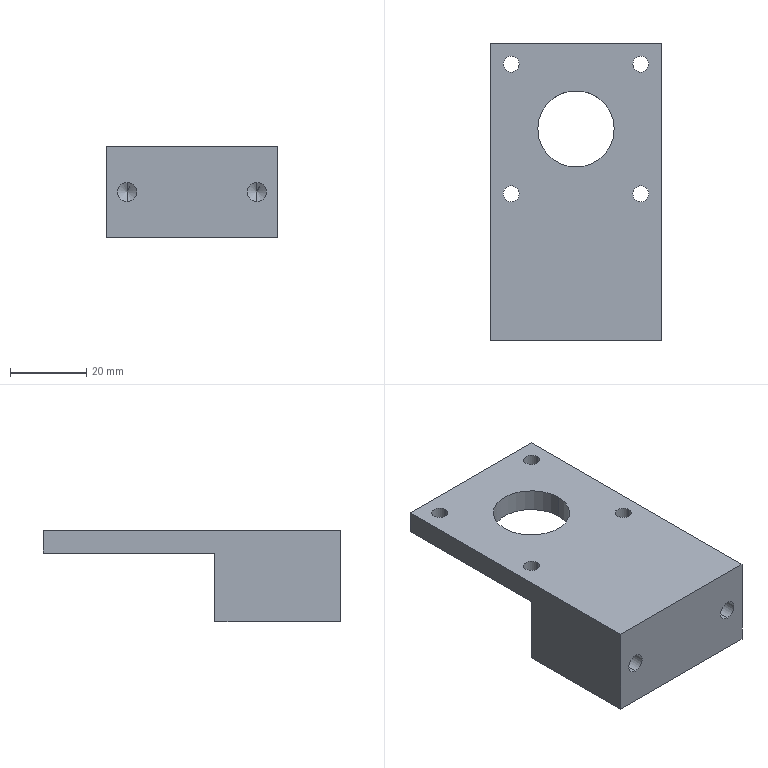Component | SolidWorks | PointedHeadDispensingCylinderSeat-2 | 1 solid | 26 faces | box 45 x 78 x 24 mm | volume 44885 mm3 | cylinder 14 | plane 8 | cone 4 | commonest cylinder face diameters 4.2 x8 5 x4 20 x2
build123d program:
from build123d import *

# Parameters (mm, degrees)
SKETCH1_W             = 45
SKETCH1_H             = 24
EXTRUDE1_DEPTH        = 33
SKETCH2_W             = 45
SKETCH2_H             = 18
EXTRUDE2_DEPTH        = 45
SKETCH3_W             = 45
SKETCH3_H             = 45
CUT_EXTRUDE1_DEPTH    = 12
M5_TAPPED_HOLE1_D     = 4.2
M5_TAPPED_HOLE1_DEPTH = 14
M5_TAPPED_HOLE1_TIP   = 1.262
SKETCH7_R             = 10
CUT_EXTRUDE2_DEPTH    = 92.831
M6_TAPPED_HOLE1_D     = 5
M6_TAPPED_HOLE1_DEPTH = 17
M6_TAPPED_HOLE1_TIP   = 1.502


with BuildPart() as part:
    # Sketch1 → Extrude1 (new body)
    with BuildSketch(Plane(origin=(0, 0, 0), x_dir=(1, 0, 0), z_dir=(0, 1, 0))):
        with Locations((22.5, -12)):
            Rectangle(SKETCH1_W, SKETCH1_H)
    extrude(amount=EXTRUDE1_DEPTH)

    # Sketch2 → Extrude2 (add)
    with BuildSketch(Plane(origin=(0, 33, 0), x_dir=(1, 0, 0), z_dir=(0, 1, 0))):
        with Locations((22.5, -9)):
            Rectangle(SKETCH2_W, SKETCH2_H)
    extrude(amount=EXTRUDE2_DEPTH)

    # Sketch3 → Cut-Extrude1 (cut)
    with BuildSketch(Plane.XY.offset(18)):
        with Locations((22.5, 55.5)):
            Rectangle(SKETCH3_W, SKETCH3_H)
    extrude(amount=-CUT_EXTRUDE1_DEPTH, mode=Mode.SUBTRACT)

    # M5 Tapped Hole1
    with Locations(Plane.XY.offset(6)):
        with Locations((5.5, 38.5), (39.5, 38.5), (39.5, 72.5), (5.5, 72.5)):
            Hole(M5_TAPPED_HOLE1_D / 2, depth=M5_TAPPED_HOLE1_DEPTH)
            with Locations((0, 0, -(M5_TAPPED_HOLE1_DEPTH + M5_TAPPED_HOLE1_TIP / 2))):  # 118° drill point
                Cone(0, M5_TAPPED_HOLE1_D / 2, M5_TAPPED_HOLE1_TIP, mode=Mode.SUBTRACT)

    # Sketch7 → Cut-Extrude2 (cut, through all)
    with BuildSketch(Plane.XY.offset(6)):
        with Locations((22.5, 55.5)):
            Circle(SKETCH7_R)
    extrude(amount=-CUT_EXTRUDE2_DEPTH, mode=Mode.SUBTRACT)

    # M6 Tapped Hole1
    with Locations(Plane.XZ):
        with Locations((5.5, 12), (39.5, 12)):
            Hole(M6_TAPPED_HOLE1_D / 2, depth=M6_TAPPED_HOLE1_DEPTH)
            with Locations((0, 0, -(M6_TAPPED_HOLE1_DEPTH + M6_TAPPED_HOLE1_TIP / 2))):  # 118° drill point
                Cone(0, M6_TAPPED_HOLE1_D / 2, M6_TAPPED_HOLE1_TIP, mode=Mode.SUBTRACT)


solid = part.part

# Placed as in the assembly
solid = solid.moved(Location((10.917, -9.628, -157.387), (-180, 0, 180)))
STEP:
#1=COLOUR_RGB('',0.7922,0.8196,0.9333);
#2=FILL_AREA_STYLE_COLOUR('',#1);
#3=FILL_AREA_STYLE('',(#2));
#4=SURFACE_STYLE_FILL_AREA(#3);
#5=SURFACE_SIDE_STYLE('',(#4));
#6=SURFACE_STYLE_USAGE(.BOTH.,#5);
#7=PRESENTATION_STYLE_ASSIGNMENT((#6));
#8=CARTESIAN_POINT('',(0.2133,0.3494,-6.669));
#9=VERTEX_POINT('',#8);
#10=CARTESIAN_POINT('',(0.2133,0.2903,-6.57));
#11=VERTEX_POINT('',#10);
#12=CARTESIAN_POINT('',(0.2133,0.2903,-6.57));
#13=DIRECTION('',(-0.,-0.515,0.8572));
#14=VECTOR('',#13,39.37);
#15=LINE('',#12,#14);
#16=EDGE_CURVE('',#9,#11,#15,.T.);
#17=ORIENTED_EDGE('',*,*,#16,.F.);
#18=CARTESIAN_POINT('',(0.2133,0.2903,-6.767));
#19=VERTEX_POINT('',#18);
#20=CARTESIAN_POINT('',(0.2133,0.2903,-6.767));
#21=DIRECTION('',(-0.,-0.515,-0.8572));
#22=VECTOR('',#21,39.37);
#23=LINE('',#20,#22);
#24=EDGE_CURVE('',#9,#19,#23,.T.);
#25=ORIENTED_EDGE('',*,*,#24,.T.);
#26=CARTESIAN_POINT('',(0.2133,0.2903,-6.669));
#27=DIRECTION('',(-0.,-1.,0.));
#28=DIRECTION('',(0.,0.,1.));
#29=AXIS2_PLACEMENT_3D('',#26,#27,#28);
#30=CIRCLE('',#29,0.09843);
#31=EDGE_CURVE('',#19,#11,#30,.T.);
#32=ORIENTED_EDGE('',*,*,#31,.T.);
#33=EDGE_LOOP('',(#17,#25,#32));
#34=FACE_OUTER_BOUND('',#33,.T.);
#35=CARTESIAN_POINT('',(0.2133,0.2903,-6.669));
#36=DIRECTION('',(-0.,-1.,0.));
#37=DIRECTION('',(0.,0.,1.));
#38=AXIS2_PLACEMENT_3D('',#35,#36,#37);
#39=CONICAL_SURFACE('',#38,0.09843,1.03);
#40=ADVANCED_FACE('',(#34),#39,.F.);
#41=ORIENTED_EDGE('',*,*,#31,.F.);
#42=CARTESIAN_POINT('',(0.2133,-0.379,-6.767));
#43=VERTEX_POINT('',#42);
#44=CARTESIAN_POINT('',(0.2133,-0.379,-6.767));
#45=DIRECTION('',(-0.,-1.,0.));
#46=VECTOR('',#45,39.37);
#47=LINE('',#44,#46);
#48=EDGE_CURVE('',#19,#43,#47,.T.);
#49=ORIENTED_EDGE('',*,*,#48,.T.);
#50=CARTESIAN_POINT('',(0.2133,-0.379,-6.57));
#51=VERTEX_POINT('',#50);
#52=CARTESIAN_POINT('',(0.2133,-0.379,-6.669));
#53=DIRECTION('',(-0.,-1.,0.));
#54=DIRECTION('',(0.,0.,1.));
#55=AXIS2_PLACEMENT_3D('',#52,#53,#54);
#56=CIRCLE('',#55,0.09843);
#57=EDGE_CURVE('',#43,#51,#56,.T.);
#58=ORIENTED_EDGE('',*,*,#57,.T.);
#59=CARTESIAN_POINT('',(0.2133,-0.379,-6.57));
#60=DIRECTION('',(-0.,-1.,0.));
#61=VECTOR('',#60,39.37);
#62=LINE('',#59,#61);
#63=EDGE_CURVE('',#11,#51,#62,.T.);
#64=ORIENTED_EDGE('',*,*,#63,.F.);
#65=EDGE_LOOP('',(#41,#49,#58,#64));
#66=FACE_OUTER_BOUND('',#65,.T.);
#67=CARTESIAN_POINT('',(0.2133,-0.379,-6.669));
#68=DIRECTION('',(-0.,-1.,0.));
#69=DIRECTION('',(0.,0.,1.));
#70=AXIS2_PLACEMENT_3D('',#67,#68,#69);
#71=CYLINDRICAL_SURFACE('',#70,0.09843);
#72=ADVANCED_FACE('',(#66),#71,.F.);
#73=CARTESIAN_POINT('',(-1.125,0.3494,-6.669));
#74=VERTEX_POINT('',#73);
#75=CARTESIAN_POINT('',(-1.125,0.2903,-6.57));
#76=VERTEX_POINT('',#75);
#77=CARTESIAN_POINT('',(-1.125,0.2903,-6.57));
#78=DIRECTION('',(-0.,-0.515,0.8572));
#79=VECTOR('',#78,39.37);
#80=LINE('',#77,#79);
#81=EDGE_CURVE('',#74,#76,#80,.T.);
#82=ORIENTED_EDGE('',*,*,#81,.F.);
#83=CARTESIAN_POINT('',(-1.125,0.2903,-6.767));
#84=VERTEX_POINT('',#83);
#85=CARTESIAN_POINT('',(-1.125,0.2903,-6.767));
#86=DIRECTION('',(-0.,-0.515,-0.8572));
#87=VECTOR('',#86,39.37);
#88=LINE('',#85,#87);
#89=EDGE_CURVE('',#74,#84,#88,.T.);
#90=ORIENTED_EDGE('',*,*,#89,.T.);
#91=CARTESIAN_POINT('',(-1.125,0.2903,-6.669));
#92=DIRECTION('',(-0.,-1.,0.));
#93=DIRECTION('',(0.,0.,1.));
#94=AXIS2_PLACEMENT_3D('',#91,#92,#93);
#95=CIRCLE('',#94,0.09843);
#96=EDGE_CURVE('',#84,#76,#95,.T.);
#97=ORIENTED_EDGE('',*,*,#96,.T.);
#98=EDGE_LOOP('',(#82,#90,#97));
#99=FACE_OUTER_BOUND('',#98,.T.);
#100=CARTESIAN_POINT('',(-1.125,0.2903,-6.669));
#101=DIRECTION('',(-0.,-1.,0.));
#102=DIRECTION('',(0.,0.,1.));
#103=AXIS2_PLACEMENT_3D('',#100,#101,#102);
#104=CONICAL_SURFACE('',#103,0.09843,1.03);
#105=ADVANCED_FACE('',(#99),#104,.F.);
#106=ORIENTED_EDGE('',*,*,#96,.F.);
#107=CARTESIAN_POINT('',(-1.125,-0.379,-6.767));
#108=VERTEX_POINT('',#107);
#109=CARTESIAN_POINT('',(-1.125,-0.379,-6.767));
#110=DIRECTION('',(-0.,-1.,0.));
#111=VECTOR('',#110,39.37);
#112=LINE('',#109,#111);
#113=EDGE_CURVE('',#84,#108,#112,.T.);
#114=ORIENTED_EDGE('',*,*,#113,.T.);
#115=CARTESIAN_POINT('',(-1.125,-0.379,-6.57));
#116=VERTEX_POINT('',#115);
#117=CARTESIAN_POINT('',(-1.125,-0.379,-6.669));
#118=DIRECTION('',(-0.,-1.,0.));
#119=DIRECTION('',(0.,0.,1.));
#120=AXIS2_PLACEMENT_3D('',#117,#118,#119);
#121=CIRCLE('',#120,0.09843);
#122=EDGE_CURVE('',#108,#116,#121,.T.);
#123=ORIENTED_EDGE('',*,*,#122,.T.);
#124=CARTESIAN_POINT('',(-1.125,-0.379,-6.57));
#125=DIRECTION('',(-0.,-1.,0.));
#126=VECTOR('',#125,39.37);
#127=LINE('',#124,#126);
#128=EDGE_CURVE('',#76,#116,#127,.T.);
#129=ORIENTED_EDGE('',*,*,#128,.F.);
#130=EDGE_LOOP('',(#106,#114,#123,#129));
#131=FACE_OUTER_BOUND('',#130,.T.);
#132=CARTESIAN_POINT('',(-1.125,-0.379,-6.669));
#133=DIRECTION('',(-0.,-1.,0.));
#134=DIRECTION('',(0.,0.,1.));
#135=AXIS2_PLACEMENT_3D('',#132,#133,#134);
#136=CYLINDRICAL_SURFACE('',#135,0.09843);
#137=ADVANCED_FACE('',(#131),#136,.F.);
#138=CARTESIAN_POINT('',(-0.06233,1.806,-6.196));
#139=VERTEX_POINT('',#138);
#140=CARTESIAN_POINT('',(-0.8497,1.806,-6.196));
#141=VERTEX_POINT('',#140);
#142=CARTESIAN_POINT('',(-0.456,1.806,-6.196));
#143=DIRECTION('',(0.,0.,-1.));
#144=DIRECTION('',(-1.,0.,0.));
#145=AXIS2_PLACEMENT_3D('',#142,#143,#144);
#146=CIRCLE('',#145,0.3937);
#147=EDGE_CURVE('',#139,#141,#146,.T.);
#148=ORIENTED_EDGE('',*,*,#147,.F.);
#149=CARTESIAN_POINT('',(-0.06233,1.806,-6.433));
#150=VERTEX_POINT('',#149);
#151=CARTESIAN_POINT('',(-0.06233,1.806,-6.196));
#152=DIRECTION('',(0.,0.,-1.));
#153=VECTOR('',#152,39.37);
#154=LINE('',#151,#153);
#155=EDGE_CURVE('',#139,#150,#154,.T.);
#156=ORIENTED_EDGE('',*,*,#155,.T.);
#157=CARTESIAN_POINT('',(-0.8497,1.806,-6.433));
#158=VERTEX_POINT('',#157);
#159=CARTESIAN_POINT('',(-0.456,1.806,-6.433));
#160=DIRECTION('',(0.,0.,-1.));
#161=DIRECTION('',(-1.,0.,0.));
#162=AXIS2_PLACEMENT_3D('',#159,#160,#161);
#163=CIRCLE('',#162,0.3937);
#164=EDGE_CURVE('',#150,#158,#163,.T.);
#165=ORIENTED_EDGE('',*,*,#164,.T.);
#166=CARTESIAN_POINT('',(-0.8497,1.806,-6.196));
#167=DIRECTION('',(0.,0.,-1.));
#168=VECTOR('',#167,39.37);
#169=LINE('',#166,#168);
#170=EDGE_CURVE('',#141,#158,#169,.T.);
#171=ORIENTED_EDGE('',*,*,#170,.F.);
#172=EDGE_LOOP('',(#148,#156,#165,#171));
#173=FACE_OUTER_BOUND('',#172,.T.);
#174=CARTESIAN_POINT('',(-0.456,1.806,-6.196));
#175=DIRECTION('',(0.,0.,-1.));
#176=DIRECTION('',(-1.,0.,0.));
#177=AXIS2_PLACEMENT_3D('',#174,#175,#176);
#178=CYLINDRICAL_SURFACE('',#177,0.3937);
#179=ADVANCED_FACE('',(#173),#178,.F.);
#180=CARTESIAN_POINT('',(0.2959,1.137,-6.196));
#181=VERTEX_POINT('',#180);
#182=CARTESIAN_POINT('',(0.1306,1.137,-6.196));
#183=VERTEX_POINT('',#182);
#184=CARTESIAN_POINT('',(0.2133,1.137,-6.196));
#185=DIRECTION('',(0.,0.,-1.));
#186=DIRECTION('',(-1.,0.,0.));
#187=AXIS2_PLACEMENT_3D('',#184,#185,#186);
#188=CIRCLE('',#187,0.08268);
#189=EDGE_CURVE('',#181,#183,#188,.T.);
#190=ORIENTED_EDGE('',*,*,#189,.F.);
#191=CARTESIAN_POINT('',(0.2959,1.137,-6.433));
#192=VERTEX_POINT('',#191);
#193=CARTESIAN_POINT('',(0.2959,1.137,-6.433));
#194=DIRECTION('',(0.,0.,-1.));
#195=VECTOR('',#194,39.37);
#196=LINE('',#193,#195);
#197=EDGE_CURVE('',#181,#192,#196,.T.);
#198=ORIENTED_EDGE('',*,*,#197,.T.);
#199=CARTESIAN_POINT('',(0.1306,1.137,-6.433));
#200=VERTEX_POINT('',#199);
#201=CARTESIAN_POINT('',(0.2133,1.137,-6.433));
#202=DIRECTION('',(0.,0.,-1.));
#203=DIRECTION('',(-1.,0.,0.));
#204=AXIS2_PLACEMENT_3D('',#201,#202,#203);
#205=CIRCLE('',#204,0.08268);
#206=EDGE_CURVE('',#192,#200,#205,.T.);
#207=ORIENTED_EDGE('',*,*,#206,.T.);
#208=CARTESIAN_POINT('',(0.1306,1.137,-6.433));
#209=DIRECTION('',(0.,0.,-1.));
#210=VECTOR('',#209,39.37);
#211=LINE('',#208,#210);
#212=EDGE_CURVE('',#183,#200,#211,.T.);
#213=ORIENTED_EDGE('',*,*,#212,.F.);
#214=EDGE_LOOP('',(#190,#198,#207,#213));
#215=FACE_OUTER_BOUND('',#214,.T.);
#216=CARTESIAN_POINT('',(0.2133,1.137,-6.433));
#217=DIRECTION('',(0.,0.,-1.));
#218=DIRECTION('',(-1.,0.,0.));
#219=AXIS2_PLACEMENT_3D('',#216,#217,#218);
#220=CYLINDRICAL_SURFACE('',#219,0.08268);
#221=ADVANCED_FACE('',(#215),#220,.F.);
#222=CARTESIAN_POINT('',(-1.043,1.137,-6.196));
#223=VERTEX_POINT('',#222);
#224=CARTESIAN_POINT('',(-1.208,1.137,-6.196));
#225=VERTEX_POINT('',#224);
#226=CARTESIAN_POINT('',(-1.125,1.137,-6.196));
#227=DIRECTION('',(0.,0.,-1.));
#228=DIRECTION('',(-1.,0.,0.));
#229=AXIS2_PLACEMENT_3D('',#226,#227,#228);
#230=CIRCLE('',#229,0.08268);
#231=EDGE_CURVE('',#223,#225,#230,.T.);
#232=ORIENTED_EDGE('',*,*,#231,.F.);
#233=CARTESIAN_POINT('',(-1.043,1.137,-6.433));
#234=VERTEX_POINT('',#233);
#235=CARTESIAN_POINT('',(-1.043,1.137,-6.433));
#236=DIRECTION('',(0.,0.,-1.));
#237=VECTOR('',#236,39.37);
#238=LINE('',#235,#237);
#239=EDGE_CURVE('',#223,#234,#238,.T.);
#240=ORIENTED_EDGE('',*,*,#239,.T.);
#241=CARTESIAN_POINT('',(-1.208,1.137,-6.433));
#242=VERTEX_POINT('',#241);
#243=CARTESIAN_POINT('',(-1.125,1.137,-6.433));
#244=DIRECTION('',(0.,0.,-1.));
#245=DIRECTION('',(-1.,0.,0.));
#246=AXIS2_PLACEMENT_3D('',#243,#244,#245);
#247=CIRCLE('',#246,0.08268);
#248=EDGE_CURVE('',#234,#242,#247,.T.);
#249=ORIENTED_EDGE('',*,*,#248,.T.);
#250=CARTESIAN_POINT('',(-1.208,1.137,-6.433));
#251=DIRECTION('',(0.,0.,-1.));
#252=VECTOR('',#251,39.37);
#253=LINE('',#250,#252);
#254=EDGE_CURVE('',#225,#242,#253,.T.);
#255=ORIENTED_EDGE('',*,*,#254,.F.);
#256=EDGE_LOOP('',(#232,#240,#249,#255));
#257=FACE_OUTER_BOUND('',#256,.T.);
#258=CARTESIAN_POINT('',(-1.125,1.137,-6.433));
#259=DIRECTION('',(0.,0.,-1.));
#260=DIRECTION('',(-1.,0.,0.));
#261=AXIS2_PLACEMENT_3D('',#258,#259,#260);
#262=CYLINDRICAL_SURFACE('',#261,0.08268);
#263=ADVANCED_FACE('',(#257),#262,.F.);
#264=CARTESIAN_POINT('',(-1.043,2.475,-6.196));
#265=VERTEX_POINT('',#264);
#266=CARTESIAN_POINT('',(-1.208,2.475,-6.196));
#267=VERTEX_POINT('',#266);
#268=CARTESIAN_POINT('',(-1.125,2.475,-6.196));
#269=DIRECTION('',(0.,0.,-1.));
#270=DIRECTION('',(-1.,0.,0.));
#271=AXIS2_PLACEMENT_3D('',#268,#269,#270);
#272=CIRCLE('',#271,0.08268);
#273=EDGE_CURVE('',#265,#267,#272,.T.);
#274=ORIENTED_EDGE('',*,*,#273,.F.);
#275=CARTESIAN_POINT('',(-1.043,2.475,-6.433));
#276=VERTEX_POINT('',#275);
#277=CARTESIAN_POINT('',(-1.043,2.475,-6.433));
#278=DIRECTION('',(0.,0.,-1.));
#279=VECTOR('',#278,39.37);
#280=LINE('',#277,#279);
#281=EDGE_CURVE('',#265,#276,#280,.T.);
#282=ORIENTED_EDGE('',*,*,#281,.T.);
#283=CARTESIAN_POINT('',(-1.208,2.475,-6.433));
#284=VERTEX_POINT('',#283);
#285=CARTESIAN_POINT('',(-1.125,2.475,-6.433));
#286=DIRECTION('',(0.,0.,-1.));
#287=DIRECTION('',(-1.,0.,0.));
#288=AXIS2_PLACEMENT_3D('',#285,#286,#287);
#289=CIRCLE('',#288,0.08268);
#290=EDGE_CURVE('',#276,#284,#289,.T.);
#291=ORIENTED_EDGE('',*,*,#290,.T.);
#292=CARTESIAN_POINT('',(-1.208,2.475,-6.433));
#293=DIRECTION('',(0.,0.,-1.));
#294=VECTOR('',#293,39.37);
#295=LINE('',#292,#294);
#296=EDGE_CURVE('',#267,#284,#295,.T.);
#297=ORIENTED_EDGE('',*,*,#296,.F.);
#298=EDGE_LOOP('',(#274,#282,#291,#297));
#299=FACE_OUTER_BOUND('',#298,.T.);
#300=CARTESIAN_POINT('',(-1.125,2.475,-6.433));
#301=DIRECTION('',(0.,0.,-1.));
#302=DIRECTION('',(-1.,0.,0.));
#303=AXIS2_PLACEMENT_3D('',#300,#301,#302);
#304=CYLINDRICAL_SURFACE('',#303,0.08268);
#305=ADVANCED_FACE('',(#299),#304,.F.);
#306=CARTESIAN_POINT('',(0.2959,2.475,-6.196));
#307=VERTEX_POINT('',#306);
#308=CARTESIAN_POINT('',(0.1306,2.475,-6.196));
#309=VERTEX_POINT('',#308);
#310=CARTESIAN_POINT('',(0.2133,2.475,-6.196));
#311=DIRECTION('',(0.,0.,-1.));
#312=DIRECTION('',(-1.,0.,0.));
#313=AXIS2_PLACEMENT_3D('',#310,#311,#312);
#314=CIRCLE('',#313,0.08268);
#315=EDGE_CURVE('',#307,#309,#314,.T.);
#316=ORIENTED_EDGE('',*,*,#315,.F.);
#317=CARTESIAN_POINT('',(0.2959,2.475,-6.433));
#318=VERTEX_POINT('',#317);
#319=CARTESIAN_POINT('',(0.2959,2.475,-6.433));
#320=DIRECTION('',(0.,0.,-1.));
#321=VECTOR('',#320,39.37);
#322=LINE('',#319,#321);
#323=EDGE_CURVE('',#307,#318,#322,.T.);
#324=ORIENTED_EDGE('',*,*,#323,.T.);
#325=CARTESIAN_POINT('',(0.1306,2.475,-6.433));
#326=VERTEX_POINT('',#325);
#327=CARTESIAN_POINT('',(0.2133,2.475,-6.433));
#328=DIRECTION('',(0.,0.,-1.));
#329=DIRECTION('',(-1.,0.,0.));
#330=AXIS2_PLACEMENT_3D('',#327,#328,#329);
#331=CIRCLE('',#330,0.08268);
#332=EDGE_CURVE('',#318,#326,#331,.T.);
#333=ORIENTED_EDGE('',*,*,#332,.T.);
#334=CARTESIAN_POINT('',(0.1306,2.475,-6.433));
#335=DIRECTION('',(0.,0.,-1.));
#336=VECTOR('',#335,39.37);
#337=LINE('',#334,#336);
#338=EDGE_CURVE('',#309,#326,#337,.T.);
#339=ORIENTED_EDGE('',*,*,#338,.F.);
#340=EDGE_LOOP('',(#316,#324,#333,#339));
#341=FACE_OUTER_BOUND('',#340,.T.);
#342=CARTESIAN_POINT('',(0.2133,2.475,-6.433));
#343=DIRECTION('',(0.,0.,-1.));
#344=DIRECTION('',(-1.,0.,0.));
#345=AXIS2_PLACEMENT_3D('',#342,#343,#344);
#346=CYLINDRICAL_SURFACE('',#345,0.08268);
#347=ADVANCED_FACE('',(#341),#346,.F.);
#348=CARTESIAN_POINT('',(0.4298,2.692,-6.196));
#349=VERTEX_POINT('',#348);
#350=CARTESIAN_POINT('',(0.4298,2.692,-6.433));
#351=VERTEX_POINT('',#350);
#352=CARTESIAN_POINT('',(0.4298,2.692,-6.196));
#353=DIRECTION('',(-0.,0.,-1.));
#354=VECTOR('',#353,39.37);
#355=LINE('',#352,#354);
#356=EDGE_CURVE('',#349,#351,#355,.T.);
#357=ORIENTED_EDGE('',*,*,#356,.T.);
#358=CARTESIAN_POINT('',(-1.342,2.692,-6.433));
#359=VERTEX_POINT('',#358);
#360=CARTESIAN_POINT('',(0.4298,2.692,-6.433));
#361=DIRECTION('',(1.,-0.,0.));
#362=VECTOR('',#361,39.37);
#363=LINE('',#360,#362);
#364=EDGE_CURVE('',#359,#351,#363,.T.);
#365=ORIENTED_EDGE('',*,*,#364,.F.);
#366=CARTESIAN_POINT('',(-1.342,2.692,-6.196));
#367=VERTEX_POINT('',#366);
#368=CARTESIAN_POINT('',(-1.342,2.692,-6.196));
#369=DIRECTION('',(-0.,-0.,1.));
#370=VECTOR('',#369,39.37);
#371=LINE('',#368,#370);
#372=EDGE_CURVE('',#359,#367,#371,.T.);
#373=ORIENTED_EDGE('',*,*,#372,.T.);
#374=CARTESIAN_POINT('',(0.4298,2.692,-6.196));
#375=DIRECTION('',(1.,-0.,0.));
#376=VECTOR('',#375,39.37);
#377=LINE('',#374,#376);
#378=EDGE_CURVE('',#367,#349,#377,.T.);
#379=ORIENTED_EDGE('',*,*,#378,.T.);
#380=EDGE_LOOP('',(#357,#365,#373,#379));
#381=FACE_OUTER_BOUND('',#380,.T.);
#382=CARTESIAN_POINT('',(0.4298,2.692,-6.905));
#383=DIRECTION('',(0.,1.,0.));
#384=DIRECTION('',(0.,0.,-1.));
#385=AXIS2_PLACEMENT_3D('',#382,#383,#384);
#386=PLANE('',#385);
#387=ADVANCED_FACE('',(#381),#386,.T.);
#388=CARTESIAN_POINT('',(0.4298,0.9202,-6.433));
#389=VERTEX_POINT('',#388);
#390=CARTESIAN_POINT('',(0.4298,0.9202,-7.141));
#391=VERTEX_POINT('',#390);
#392=CARTESIAN_POINT('',(0.4298,0.9202,-6.196));
#393=DIRECTION('',(-0.,0.,-1.));
#394=VECTOR('',#393,39.37);
#395=LINE('',#392,#394);
#396=EDGE_CURVE('',#389,#391,#395,.T.);
#397=ORIENTED_EDGE('',*,*,#396,.F.);
#398=CARTESIAN_POINT('',(0.4298,2.692,-6.433));
#399=DIRECTION('',(-0.,-1.,-0.));
#400=VECTOR('',#399,39.37);
#401=LINE('',#398,#400);
#402=EDGE_CURVE('',#351,#389,#401,.T.);
#403=ORIENTED_EDGE('',*,*,#402,.F.);
#404=ORIENTED_EDGE('',*,*,#356,.F.);
#405=CARTESIAN_POINT('',(0.4298,-0.379,-6.196));
#406=VERTEX_POINT('',#405);
#407=CARTESIAN_POINT('',(0.4298,0.9202,-6.196));
#408=DIRECTION('',(-0.,-1.,0.));
#409=VECTOR('',#408,39.37);
#410=LINE('',#407,#409);
#411=EDGE_CURVE('',#349,#406,#410,.T.);
#412=ORIENTED_EDGE('',*,*,#411,.T.);
#413=CARTESIAN_POINT('',(0.4298,-0.379,-7.141));
#414=VERTEX_POINT('',#413);
#415=CARTESIAN_POINT('',(0.4298,-0.379,-6.196));
#416=DIRECTION('',(-0.,0.,-1.));
#417=VECTOR('',#416,39.37);
#418=LINE('',#415,#417);
#419=EDGE_CURVE('',#406,#414,#418,.T.);
#420=ORIENTED_EDGE('',*,*,#419,.T.);
#421=CARTESIAN_POINT('',(0.4298,0.9202,-7.141));
#422=DIRECTION('',(-0.,-1.,0.));
#423=VECTOR('',#422,39.37);
#424=LINE('',#421,#423);
#425=EDGE_CURVE('',#391,#414,#424,.T.);
#426=ORIENTED_EDGE('',*,*,#425,.F.);
#427=EDGE_LOOP('',(#397,#403,#404,#412,#420,#426));
#428=FACE_OUTER_BOUND('',#427,.T.);
#429=CARTESIAN_POINT('',(0.4298,0.9202,-6.196));
#430=DIRECTION('',(-1.,0.,0.));
#431=DIRECTION('',(0.,-0.,1.));
#432=AXIS2_PLACEMENT_3D('',#429,#430,#431);
#433=PLANE('',#432);
#434=ADVANCED_FACE('',(#428),#433,.F.);
#435=CARTESIAN_POINT('',(-1.342,-0.379,-7.141));
#436=VERTEX_POINT('',#435);
#437=CARTESIAN_POINT('',(0.4298,-0.379,-7.141));
#438=DIRECTION('',(-1.,0.,-0.));
#439=VECTOR('',#438,39.37);
#440=LINE('',#437,#439);
#441=EDGE_CURVE('',#414,#436,#440,.T.);
#442=ORIENTED_EDGE('',*,*,#441,.T.);
#443=CARTESIAN_POINT('',(-1.342,0.9202,-7.141));
#444=VERTEX_POINT('',#443);
#445=CARTESIAN_POINT('',(-1.342,0.9202,-7.141));
#446=DIRECTION('',(-0.,-1.,0.));
#447=VECTOR('',#446,39.37);
#448=LINE('',#445,#447);
#449=EDGE_CURVE('',#444,#436,#448,.T.);
#450=ORIENTED_EDGE('',*,*,#449,.F.);
#451=CARTESIAN_POINT('',(0.4298,0.9202,-7.141));
#452=DIRECTION('',(-1.,0.,-0.));
#453=VECTOR('',#452,39.37);
#454=LINE('',#451,#453);
#455=EDGE_CURVE('',#391,#444,#454,.T.);
#456=ORIENTED_EDGE('',*,*,#455,.F.);
#457=ORIENTED_EDGE('',*,*,#425,.T.);
#458=EDGE_LOOP('',(#442,#450,#456,#457));
#459=FACE_OUTER_BOUND('',#458,.T.);
#460=CARTESIAN_POINT('',(0.4298,0.9202,-7.141));
#461=DIRECTION('',(-0.,-0.,1.));
#462=DIRECTION('',(1.,-0.,0.));
#463=AXIS2_PLACEMENT_3D('',#460,#461,#462);
#464=PLANE('',#463);
#465=ADVANCED_FACE('',(#459),#464,.F.);
#466=CARTESIAN_POINT('',(-1.342,0.9202,-6.433));
#467=VERTEX_POINT('',#466);
#468=CARTESIAN_POINT('',(-1.342,2.692,-6.433));
#469=DIRECTION('',(0.,1.,0.));
#470=VECTOR('',#469,39.37);
#471=LINE('',#468,#470);
#472=EDGE_CURVE('',#467,#359,#471,.T.);
#473=ORIENTED_EDGE('',*,*,#472,.F.);
#474=CARTESIAN_POINT('',(-1.342,0.9202,-6.196));
#475=DIRECTION('',(-0.,-0.,1.));
#476=VECTOR('',#475,39.37);
#477=LINE('',#474,#476);
#478=EDGE_CURVE('',#444,#467,#477,.T.);
#479=ORIENTED_EDGE('',*,*,#478,.F.);
#480=ORIENTED_EDGE('',*,*,#449,.T.);
#481=CARTESIAN_POINT('',(-1.342,-0.379,-6.196));
#482=VERTEX_POINT('',#481);
#483=CARTESIAN_POINT('',(-1.342,-0.379,-6.196));
#484=DIRECTION('',(-0.,-0.,1.));
#485=VECTOR('',#484,39.37);
#486=LINE('',#483,#485);
#487=EDGE_CURVE('',#436,#482,#486,.T.);
#488=ORIENTED_EDGE('',*,*,#487,.T.);
#489=CARTESIAN_POINT('',(-1.342,0.9202,-6.196));
#490=DIRECTION('',(-0.,-1.,0.));
#491=VECTOR('',#490,39.37);
#492=LINE('',#489,#491);
#493=EDGE_CURVE('',#367,#482,#492,.T.);
#494=ORIENTED_EDGE('',*,*,#493,.F.);
#495=ORIENTED_EDGE('',*,*,#372,.F.);
#496=EDGE_LOOP('',(#473,#479,#480,#488,#494,#495));
#497=FACE_OUTER_BOUND('',#496,.T.);
#498=CARTESIAN_POINT('',(-1.342,0.9202,-6.196));
#499=DIRECTION('',(1.,-0.,0.));
#500=DIRECTION('',(0.,0.,-1.));
#501=AXIS2_PLACEMENT_3D('',#498,#499,#500);
#502=PLANE('',#501);
#503=ADVANCED_FACE('',(#497),#502,.F.);
#504=CARTESIAN_POINT('',(-0.456,1.806,-6.196));
#505=DIRECTION('',(0.,0.,-1.));
#506=DIRECTION('',(-1.,0.,0.));
#507=AXIS2_PLACEMENT_3D('',#504,#505,#506);
#508=CIRCLE('',#507,0.3937);
#509=EDGE_CURVE('',#141,#139,#508,.T.);
#510=ORIENTED_EDGE('',*,*,#509,.T.);
#511=ORIENTED_EDGE('',*,*,#147,.T.);
#512=EDGE_LOOP('',(#510,#511));
#513=FACE_BOUND('',#512,.T.);
#514=CARTESIAN_POINT('',(0.2133,1.137,-6.196));
#515=DIRECTION('',(0.,0.,-1.));
#516=DIRECTION('',(-1.,0.,0.));
#517=AXIS2_PLACEMENT_3D('',#514,#515,#516);
#518=CIRCLE('',#517,0.08268);
#519=EDGE_CURVE('',#183,#181,#518,.T.);
#520=ORIENTED_EDGE('',*,*,#519,.T.);
#521=ORIENTED_EDGE('',*,*,#189,.T.);
#522=EDGE_LOOP('',(#520,#521));
#523=FACE_BOUND('',#522,.T.);
#524=CARTESIAN_POINT('',(-1.125,1.137,-6.196));
#525=DIRECTION('',(0.,0.,-1.));
#526=DIRECTION('',(-1.,0.,0.));
#527=AXIS2_PLACEMENT_3D('',#524,#525,#526);
#528=CIRCLE('',#527,0.08268);
#529=EDGE_CURVE('',#225,#223,#528,.T.);
#530=ORIENTED_EDGE('',*,*,#529,.T.);
#531=ORIENTED_EDGE('',*,*,#231,.T.);
#532=EDGE_LOOP('',(#530,#531));
#533=FACE_BOUND('',#532,.T.);
#534=CARTESIAN_POINT('',(-1.125,2.475,-6.196));
#535=DIRECTION('',(0.,0.,-1.));
#536=DIRECTION('',(-1.,0.,0.));
#537=AXIS2_PLACEMENT_3D('',#534,#535,#536);
#538=CIRCLE('',#537,0.08268);
#539=EDGE_CURVE('',#267,#265,#538,.T.);
#540=ORIENTED_EDGE('',*,*,#539,.T.);
#541=ORIENTED_EDGE('',*,*,#273,.T.);
#542=EDGE_LOOP('',(#540,#541));
#543=FACE_BOUND('',#542,.T.);
#544=CARTESIAN_POINT('',(0.2133,2.475,-6.196));
#545=DIRECTION('',(0.,0.,-1.));
#546=DIRECTION('',(-1.,0.,0.));
#547=AXIS2_PLACEMENT_3D('',#544,#545,#546);
#548=CIRCLE('',#547,0.08268);
#549=EDGE_CURVE('',#309,#307,#548,.T.);
#550=ORIENTED_EDGE('',*,*,#549,.T.);
#551=ORIENTED_EDGE('',*,*,#315,.T.);
#552=EDGE_LOOP('',(#550,#551));
#553=FACE_BOUND('',#552,.T.);
#554=CARTESIAN_POINT('',(0.4298,-0.379,-6.196));
#555=DIRECTION('',(1.,-0.,0.));
#556=VECTOR('',#555,39.37);
#557=LINE('',#554,#556);
#558=EDGE_CURVE('',#482,#406,#557,.T.);
#559=ORIENTED_EDGE('',*,*,#558,.T.);
#560=ORIENTED_EDGE('',*,*,#411,.F.);
#561=ORIENTED_EDGE('',*,*,#378,.F.);
#562=ORIENTED_EDGE('',*,*,#493,.T.);
#563=EDGE_LOOP('',(#559,#560,#561,#562));
#564=FACE_OUTER_BOUND('',#563,.T.);
#565=CARTESIAN_POINT('',(0.4298,0.9202,-6.196));
#566=DIRECTION('',(0.,0.,-1.));
#567=DIRECTION('',(-1.,0.,-0.));
#568=AXIS2_PLACEMENT_3D('',#565,#566,#567);
#569=PLANE('',#568);
#570=ADVANCED_FACE('',(#513,#523,#533,#543,#553,#564),#569,.F.);
#571=ORIENTED_EDGE('',*,*,#478,.T.);
#572=CARTESIAN_POINT('',(0.4298,0.9202,-6.433));
#573=DIRECTION('',(-1.,0.,-0.));
#574=VECTOR('',#573,39.37);
#575=LINE('',#572,#574);
#576=EDGE_CURVE('',#389,#467,#575,.T.);
#577=ORIENTED_EDGE('',*,*,#576,.F.);
#578=ORIENTED_EDGE('',*,*,#396,.T.);
#579=ORIENTED_EDGE('',*,*,#455,.T.);
#580=EDGE_LOOP('',(#571,#577,#578,#579));
#581=FACE_OUTER_BOUND('',#580,.T.);
#582=CARTESIAN_POINT('',(0.4298,0.9202,-7.141));
#583=DIRECTION('',(0.,1.,0.));
#584=DIRECTION('',(0.,0.,-1.));
#585=AXIS2_PLACEMENT_3D('',#582,#583,#584);
#586=PLANE('',#585);
#587=ADVANCED_FACE('',(#581),#586,.T.);
#588=CARTESIAN_POINT('',(0.2133,-0.379,-6.669));
#589=DIRECTION('',(-0.,-1.,0.));
#590=DIRECTION('',(0.,0.,1.));
#591=AXIS2_PLACEMENT_3D('',#588,#589,#590);
#592=CIRCLE('',#591,0.09843);
#593=EDGE_CURVE('',#51,#43,#592,.T.);
#594=ORIENTED_EDGE('',*,*,#593,.F.);
#595=ORIENTED_EDGE('',*,*,#57,.F.);
#596=EDGE_LOOP('',(#594,#595));
#597=FACE_BOUND('',#596,.T.);
#598=CARTESIAN_POINT('',(-1.125,-0.379,-6.669));
#599=DIRECTION('',(-0.,-1.,0.));
#600=DIRECTION('',(0.,0.,1.));
#601=AXIS2_PLACEMENT_3D('',#598,#599,#600);
#602=CIRCLE('',#601,0.09843);
#603=EDGE_CURVE('',#116,#108,#602,.T.);
#604=ORIENTED_EDGE('',*,*,#603,.F.);
#605=ORIENTED_EDGE('',*,*,#122,.F.);
#606=EDGE_LOOP('',(#604,#605));
#607=FACE_BOUND('',#606,.T.);
#608=ORIENTED_EDGE('',*,*,#419,.F.);
#609=ORIENTED_EDGE('',*,*,#558,.F.);
#610=ORIENTED_EDGE('',*,*,#487,.F.);
#611=ORIENTED_EDGE('',*,*,#441,.F.);
#612=EDGE_LOOP('',(#608,#609,#610,#611));
#613=FACE_OUTER_BOUND('',#612,.T.);
#614=CARTESIAN_POINT('',(0.4298,-0.379,-7.141));
#615=DIRECTION('',(0.,1.,0.));
#616=DIRECTION('',(0.,0.,-1.));
#617=AXIS2_PLACEMENT_3D('',#614,#615,#616);
#618=PLANE('',#617);
#619=ADVANCED_FACE('',(#597,#607,#613),#618,.F.);
#620=CARTESIAN_POINT('',(-0.456,1.806,-6.433));
#621=DIRECTION('',(0.,0.,-1.));
#622=DIRECTION('',(-1.,0.,0.));
#623=AXIS2_PLACEMENT_3D('',#620,#621,#622);
#624=CIRCLE('',#623,0.3937);
#625=EDGE_CURVE('',#158,#150,#624,.T.);
#626=ORIENTED_EDGE('',*,*,#625,.F.);
#627=ORIENTED_EDGE('',*,*,#164,.F.);
#628=EDGE_LOOP('',(#626,#627));
#629=FACE_BOUND('',#628,.T.);
#630=CARTESIAN_POINT('',(0.2133,1.137,-6.433));
#631=DIRECTION('',(0.,0.,-1.));
#632=DIRECTION('',(-1.,0.,0.));
#633=AXIS2_PLACEMENT_3D('',#630,#631,#632);
#634=CIRCLE('',#633,0.08268);
#635=EDGE_CURVE('',#200,#192,#634,.T.);
#636=ORIENTED_EDGE('',*,*,#635,.F.);
#637=ORIENTED_EDGE('',*,*,#206,.F.);
#638=EDGE_LOOP('',(#636,#637));
#639=FACE_BOUND('',#638,.T.);
#640=CARTESIAN_POINT('',(-1.125,1.137,-6.433));
#641=DIRECTION('',(0.,0.,-1.));
#642=DIRECTION('',(-1.,0.,0.));
#643=AXIS2_PLACEMENT_3D('',#640,#641,#642);
#644=CIRCLE('',#643,0.08268);
#645=EDGE_CURVE('',#242,#234,#644,.T.);
#646=ORIENTED_EDGE('',*,*,#645,.F.);
#647=ORIENTED_EDGE('',*,*,#248,.F.);
#648=EDGE_LOOP('',(#646,#647));
#649=FACE_BOUND('',#648,.T.);
#650=CARTESIAN_POINT('',(-1.125,2.475,-6.433));
#651=DIRECTION('',(0.,0.,-1.));
#652=DIRECTION('',(-1.,0.,0.));
#653=AXIS2_PLACEMENT_3D('',#650,#651,#652);
#654=CIRCLE('',#653,0.08268);
#655=EDGE_CURVE('',#284,#276,#654,.T.);
#656=ORIENTED_EDGE('',*,*,#655,.F.);
#657=ORIENTED_EDGE('',*,*,#290,.F.);
#658=EDGE_LOOP('',(#656,#657));
#659=FACE_BOUND('',#658,.T.);
#660=CARTESIAN_POINT('',(0.2133,2.475,-6.433));
#661=DIRECTION('',(0.,0.,-1.));
#662=DIRECTION('',(-1.,0.,0.));
#663=AXIS2_PLACEMENT_3D('',#660,#661,#662);
#664=CIRCLE('',#663,0.08268);
#665=EDGE_CURVE('',#326,#318,#664,.T.);
#666=ORIENTED_EDGE('',*,*,#665,.F.);
#667=ORIENTED_EDGE('',*,*,#332,.F.);
#668=EDGE_LOOP('',(#666,#667));
#669=FACE_BOUND('',#668,.T.);
#670=ORIENTED_EDGE('',*,*,#402,.T.);
#671=ORIENTED_EDGE('',*,*,#576,.T.);
#672=ORIENTED_EDGE('',*,*,#472,.T.);
#673=ORIENTED_EDGE('',*,*,#364,.T.);
#674=EDGE_LOOP('',(#670,#671,#672,#673));
#675=FACE_OUTER_BOUND('',#674,.T.);
#676=CARTESIAN_POINT('',(0.4298,0.9202,-6.433));
#677=DIRECTION('',(0.,0.,-1.));
#678=DIRECTION('',(-1.,0.,-0.));
#679=AXIS2_PLACEMENT_3D('',#676,#677,#678);
#680=PLANE('',#679);
#681=ADVANCED_FACE('',(#629,#639,#649,#659,#669,#675),#680,.T.);
#682=ORIENTED_EDGE('',*,*,#323,.F.);
#683=ORIENTED_EDGE('',*,*,#549,.F.);
#684=ORIENTED_EDGE('',*,*,#338,.T.);
#685=ORIENTED_EDGE('',*,*,#665,.T.);
#686=EDGE_LOOP('',(#682,#683,#684,#685));
#687=FACE_OUTER_BOUND('',#686,.T.);
#688=CARTESIAN_POINT('',(0.2133,2.475,-6.433));
#689=DIRECTION('',(0.,0.,-1.));
#690=DIRECTION('',(-1.,0.,0.));
#691=AXIS2_PLACEMENT_3D('',#688,#689,#690);
#692=CYLINDRICAL_SURFACE('',#691,0.08268);
#693=ADVANCED_FACE('',(#687),#692,.F.);
#694=ORIENTED_EDGE('',*,*,#281,.F.);
#695=ORIENTED_EDGE('',*,*,#539,.F.);
#696=ORIENTED_EDGE('',*,*,#296,.T.);
#697=ORIENTED_EDGE('',*,*,#655,.T.);
#698=EDGE_LOOP('',(#694,#695,#696,#697));
#699=FACE_OUTER_BOUND('',#698,.T.);
#700=CARTESIAN_POINT('',(-1.125,2.475,-6.433));
#701=DIRECTION('',(0.,0.,-1.));
#702=DIRECTION('',(-1.,0.,0.));
#703=AXIS2_PLACEMENT_3D('',#700,#701,#702);
#704=CYLINDRICAL_SURFACE('',#703,0.08268);
#705=ADVANCED_FACE('',(#699),#704,.F.);
#706=ORIENTED_EDGE('',*,*,#239,.F.);
#707=ORIENTED_EDGE('',*,*,#529,.F.);
#708=ORIENTED_EDGE('',*,*,#254,.T.);
#709=ORIENTED_EDGE('',*,*,#645,.T.);
#710=EDGE_LOOP('',(#706,#707,#708,#709));
#711=FACE_OUTER_BOUND('',#710,.T.);
#712=CARTESIAN_POINT('',(-1.125,1.137,-6.433));
#713=DIRECTION('',(0.,0.,-1.));
#714=DIRECTION('',(-1.,0.,0.));
#715=AXIS2_PLACEMENT_3D('',#712,#713,#714);
#716=CYLINDRICAL_SURFACE('',#715,0.08268);
#717=ADVANCED_FACE('',(#711),#716,.F.);
#718=ORIENTED_EDGE('',*,*,#197,.F.);
#719=ORIENTED_EDGE('',*,*,#519,.F.);
#720=ORIENTED_EDGE('',*,*,#212,.T.);
#721=ORIENTED_EDGE('',*,*,#635,.T.);
#722=EDGE_LOOP('',(#718,#719,#720,#721));
#723=FACE_OUTER_BOUND('',#722,.T.);
#724=CARTESIAN_POINT('',(0.2133,1.137,-6.433));
#725=DIRECTION('',(0.,0.,-1.));
#726=DIRECTION('',(-1.,0.,0.));
#727=AXIS2_PLACEMENT_3D('',#724,#725,#726);
#728=CYLINDRICAL_SURFACE('',#727,0.08268);
#729=ADVANCED_FACE('',(#723),#728,.F.);
#730=ORIENTED_EDGE('',*,*,#155,.F.);
#731=ORIENTED_EDGE('',*,*,#509,.F.);
#732=ORIENTED_EDGE('',*,*,#170,.T.);
#733=ORIENTED_EDGE('',*,*,#625,.T.);
#734=EDGE_LOOP('',(#730,#731,#732,#733));
#735=FACE_OUTER_BOUND('',#734,.T.);
#736=CARTESIAN_POINT('',(-0.456,1.806,-6.196));
#737=DIRECTION('',(0.,0.,-1.));
#738=DIRECTION('',(-1.,0.,0.));
#739=AXIS2_PLACEMENT_3D('',#736,#737,#738);
#740=CYLINDRICAL_SURFACE('',#739,0.3937);
#741=ADVANCED_FACE('',(#735),#740,.F.);
#742=ORIENTED_EDGE('',*,*,#113,.F.);
#743=CARTESIAN_POINT('',(-1.125,0.2903,-6.669));
#744=DIRECTION('',(-0.,-1.,0.));
#745=DIRECTION('',(0.,0.,1.));
#746=AXIS2_PLACEMENT_3D('',#743,#744,#745);
#747=CIRCLE('',#746,0.09843);
#748=EDGE_CURVE('',#76,#84,#747,.T.);
#749=ORIENTED_EDGE('',*,*,#748,.F.);
#750=ORIENTED_EDGE('',*,*,#128,.T.);
#751=ORIENTED_EDGE('',*,*,#603,.T.);
#752=EDGE_LOOP('',(#742,#749,#750,#751));
#753=FACE_OUTER_BOUND('',#752,.T.);
#754=CARTESIAN_POINT('',(-1.125,-0.379,-6.669));
#755=DIRECTION('',(-0.,-1.,0.));
#756=DIRECTION('',(0.,0.,1.));
#757=AXIS2_PLACEMENT_3D('',#754,#755,#756);
#758=CYLINDRICAL_SURFACE('',#757,0.09843);
#759=ADVANCED_FACE('',(#753),#758,.F.);
#760=ORIENTED_EDGE('',*,*,#89,.F.);
#761=ORIENTED_EDGE('',*,*,#81,.T.);
#762=ORIENTED_EDGE('',*,*,#748,.T.);
#763=EDGE_LOOP('',(#760,#761,#762));
#764=FACE_OUTER_BOUND('',#763,.T.);
#765=CARTESIAN_POINT('',(-1.125,0.2903,-6.669));
#766=DIRECTION('',(-0.,-1.,0.));
#767=DIRECTION('',(0.,0.,1.));
#768=AXIS2_PLACEMENT_3D('',#765,#766,#767);
#769=CONICAL_SURFACE('',#768,0.09843,1.03);
#770=ADVANCED_FACE('',(#764),#769,.F.);
#771=ORIENTED_EDGE('',*,*,#48,.F.);
#772=CARTESIAN_POINT('',(0.2133,0.2903,-6.669));
#773=DIRECTION('',(-0.,-1.,0.));
#774=DIRECTION('',(0.,0.,1.));
#775=AXIS2_PLACEMENT_3D('',#772,#773,#774);
#776=CIRCLE('',#775,0.09843);
#777=EDGE_CURVE('',#11,#19,#776,.T.);
#778=ORIENTED_EDGE('',*,*,#777,.F.);
#779=ORIENTED_EDGE('',*,*,#63,.T.);
#780=ORIENTED_EDGE('',*,*,#593,.T.);
#781=EDGE_LOOP('',(#771,#778,#779,#780));
#782=FACE_OUTER_BOUND('',#781,.T.);
#783=CARTESIAN_POINT('',(0.2133,-0.379,-6.669));
#784=DIRECTION('',(-0.,-1.,0.));
#785=DIRECTION('',(0.,0.,1.));
#786=AXIS2_PLACEMENT_3D('',#783,#784,#785);
#787=CYLINDRICAL_SURFACE('',#786,0.09843);
#788=ADVANCED_FACE('',(#782),#787,.F.);
#789=ORIENTED_EDGE('',*,*,#24,.F.);
#790=ORIENTED_EDGE('',*,*,#16,.T.);
#791=ORIENTED_EDGE('',*,*,#777,.T.);
#792=EDGE_LOOP('',(#789,#790,#791));
#793=FACE_OUTER_BOUND('',#792,.T.);
#794=CARTESIAN_POINT('',(0.2133,0.2903,-6.669));
#795=DIRECTION('',(-0.,-1.,0.));
#796=DIRECTION('',(0.,0.,1.));
#797=AXIS2_PLACEMENT_3D('',#794,#795,#796);
#798=CONICAL_SURFACE('',#797,0.09843,1.03);
#799=ADVANCED_FACE('',(#793),#798,.F.);
#800=CLOSED_SHELL('',(#40,#72,#105,#137,#179,#221,#263,#305,#347,#387,#434,#465,#503,#570,#587,#619,#681,#693,#705,#717,#729,#741,#759,#770,#788,#799));
#801=MANIFOLD_SOLID_BREP('',#800);
#802=STYLED_ITEM('',(#7),#801);
#803=PRESENTATION_LAYER_ASSIGNMENT('','',(#802));
#804=(LENGTH_UNIT()NAMED_UNIT(*)SI_UNIT($,.METRE.));
#805=LENGTH_MEASURE_WITH_UNIT(LENGTH_MEASURE(0.0254),#804);
#806=DIMENSIONAL_EXPONENTS(1.,0.,0.,0.,0.,0.,0.);
#807=(CONVERSION_BASED_UNIT('',#805)LENGTH_UNIT()NAMED_UNIT(#806));
#808=UNCERTAINTY_MEASURE_WITH_UNIT(LENGTH_MEASURE(0.00001),#807,'','');
#809=(NAMED_UNIT(*)PLANE_ANGLE_UNIT()SI_UNIT($,.RADIAN.));
#810=(NAMED_UNIT(*)SI_UNIT($,.STERADIAN.)SOLID_ANGLE_UNIT());
#811=(GEOMETRIC_REPRESENTATION_CONTEXT(3)GLOBAL_UNCERTAINTY_ASSIGNED_CONTEXT((#808))GLOBAL_UNIT_ASSIGNED_CONTEXT((#807,#809,#810))REPRESENTATION_CONTEXT('',''));
#812=MECHANICAL_DESIGN_GEOMETRIC_PRESENTATION_REPRESENTATION('',(#802),#811);
#813=CARTESIAN_POINT('',(0.,0.,0.));
#814=DIRECTION('',(0.,0.,1.));
#815=DIRECTION('',(1.,0.,0.));
#816=AXIS2_PLACEMENT_3D('',#813,#814,#815);
#817=(LENGTH_UNIT()NAMED_UNIT(*)SI_UNIT($,.METRE.));
#818=LENGTH_MEASURE_WITH_UNIT(LENGTH_MEASURE(0.0254),#817);
#819=DIMENSIONAL_EXPONENTS(1.,0.,0.,0.,0.,0.,0.);
#820=(CONVERSION_BASED_UNIT('',#818)LENGTH_UNIT()NAMED_UNIT(#819));
#821=UNCERTAINTY_MEASURE_WITH_UNIT(LENGTH_MEASURE(0.00001),#820,'','');
#822=(NAMED_UNIT(*)PLANE_ANGLE_UNIT()SI_UNIT($,.RADIAN.));
#823=(NAMED_UNIT(*)SI_UNIT($,.STERADIAN.)SOLID_ANGLE_UNIT());
#824=(GEOMETRIC_REPRESENTATION_CONTEXT(3)GLOBAL_UNCERTAINTY_ASSIGNED_CONTEXT((#821))GLOBAL_UNIT_ASSIGNED_CONTEXT((#820,#822,#823))REPRESENTATION_CONTEXT('',''));
#825=ADVANCED_BREP_SHAPE_REPRESENTATION('',(#801,#816),#824);